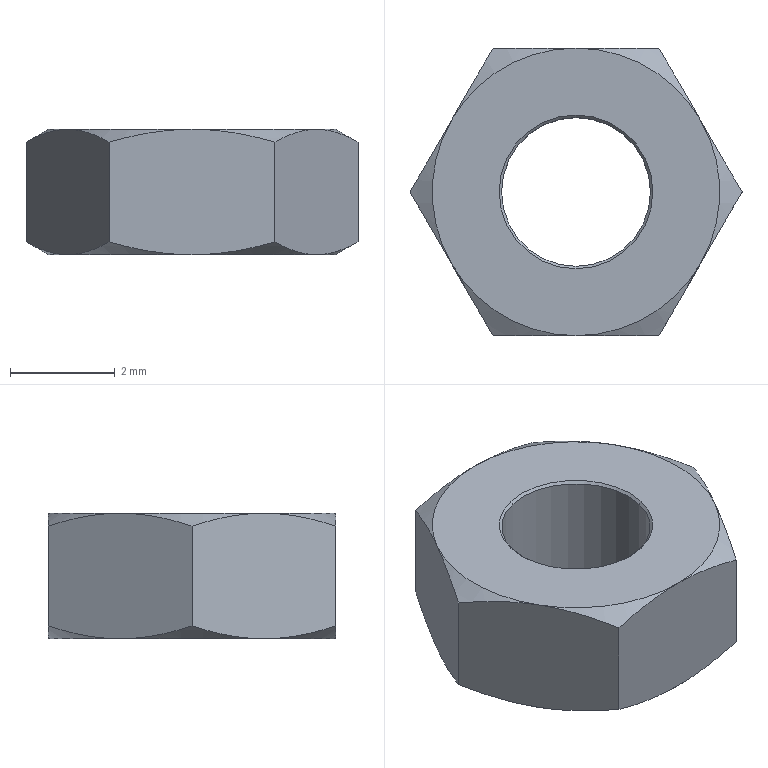Component | NX | 09_NUT | 1 solid | 23 faces | volume 47 mm3 | cone 14 | plane 8 | cylinder 1 | commonest cylinder face diameters 2.847 x1